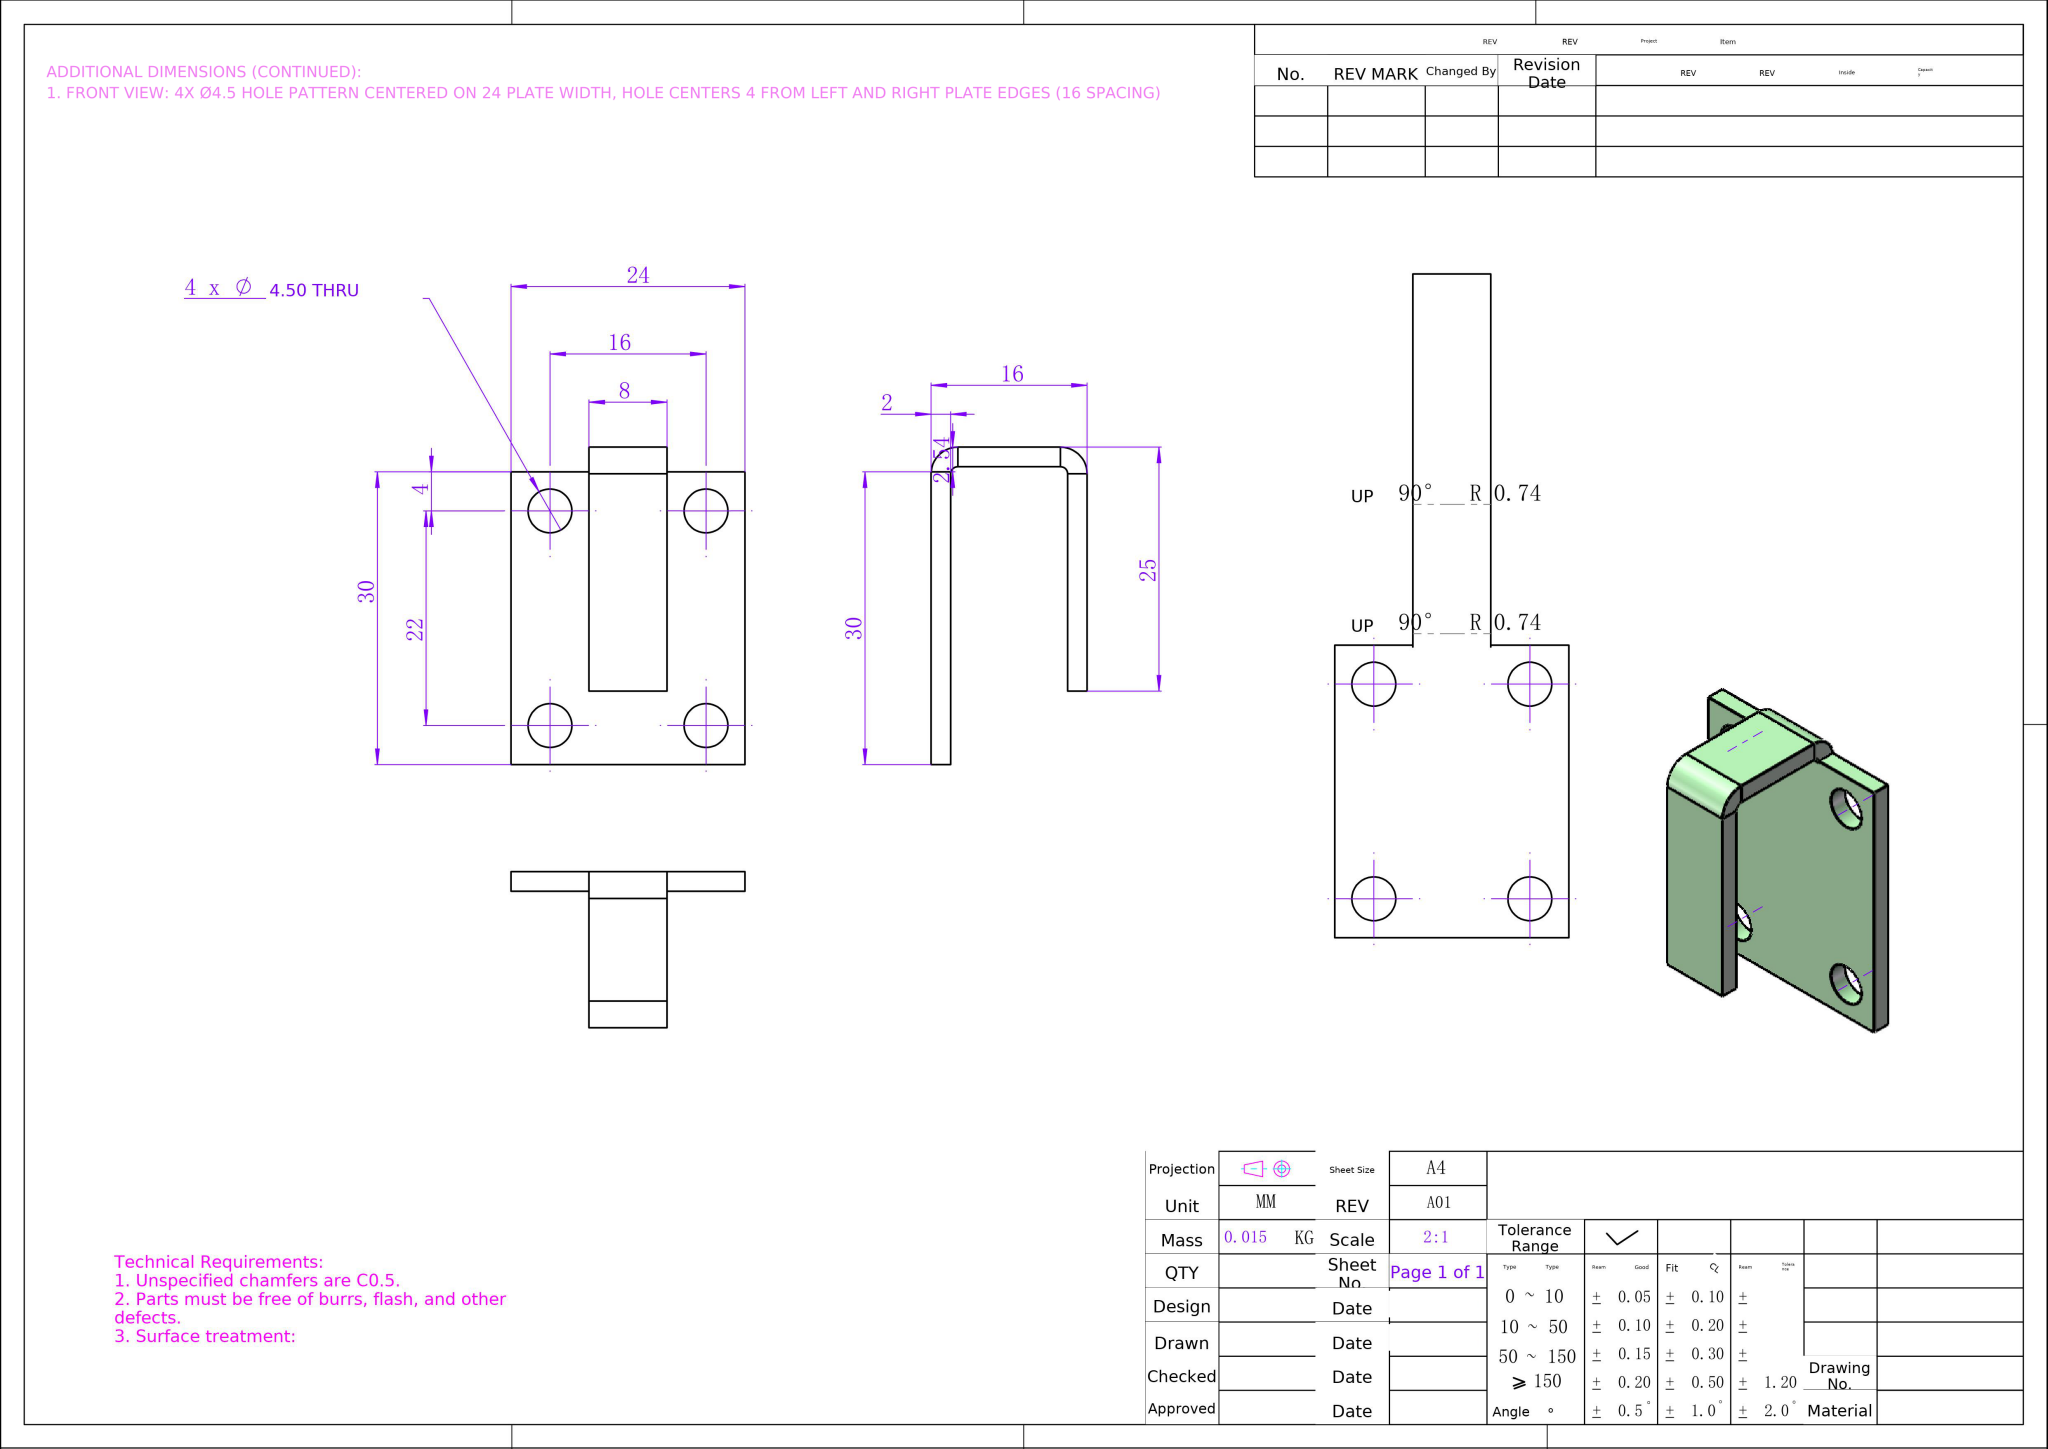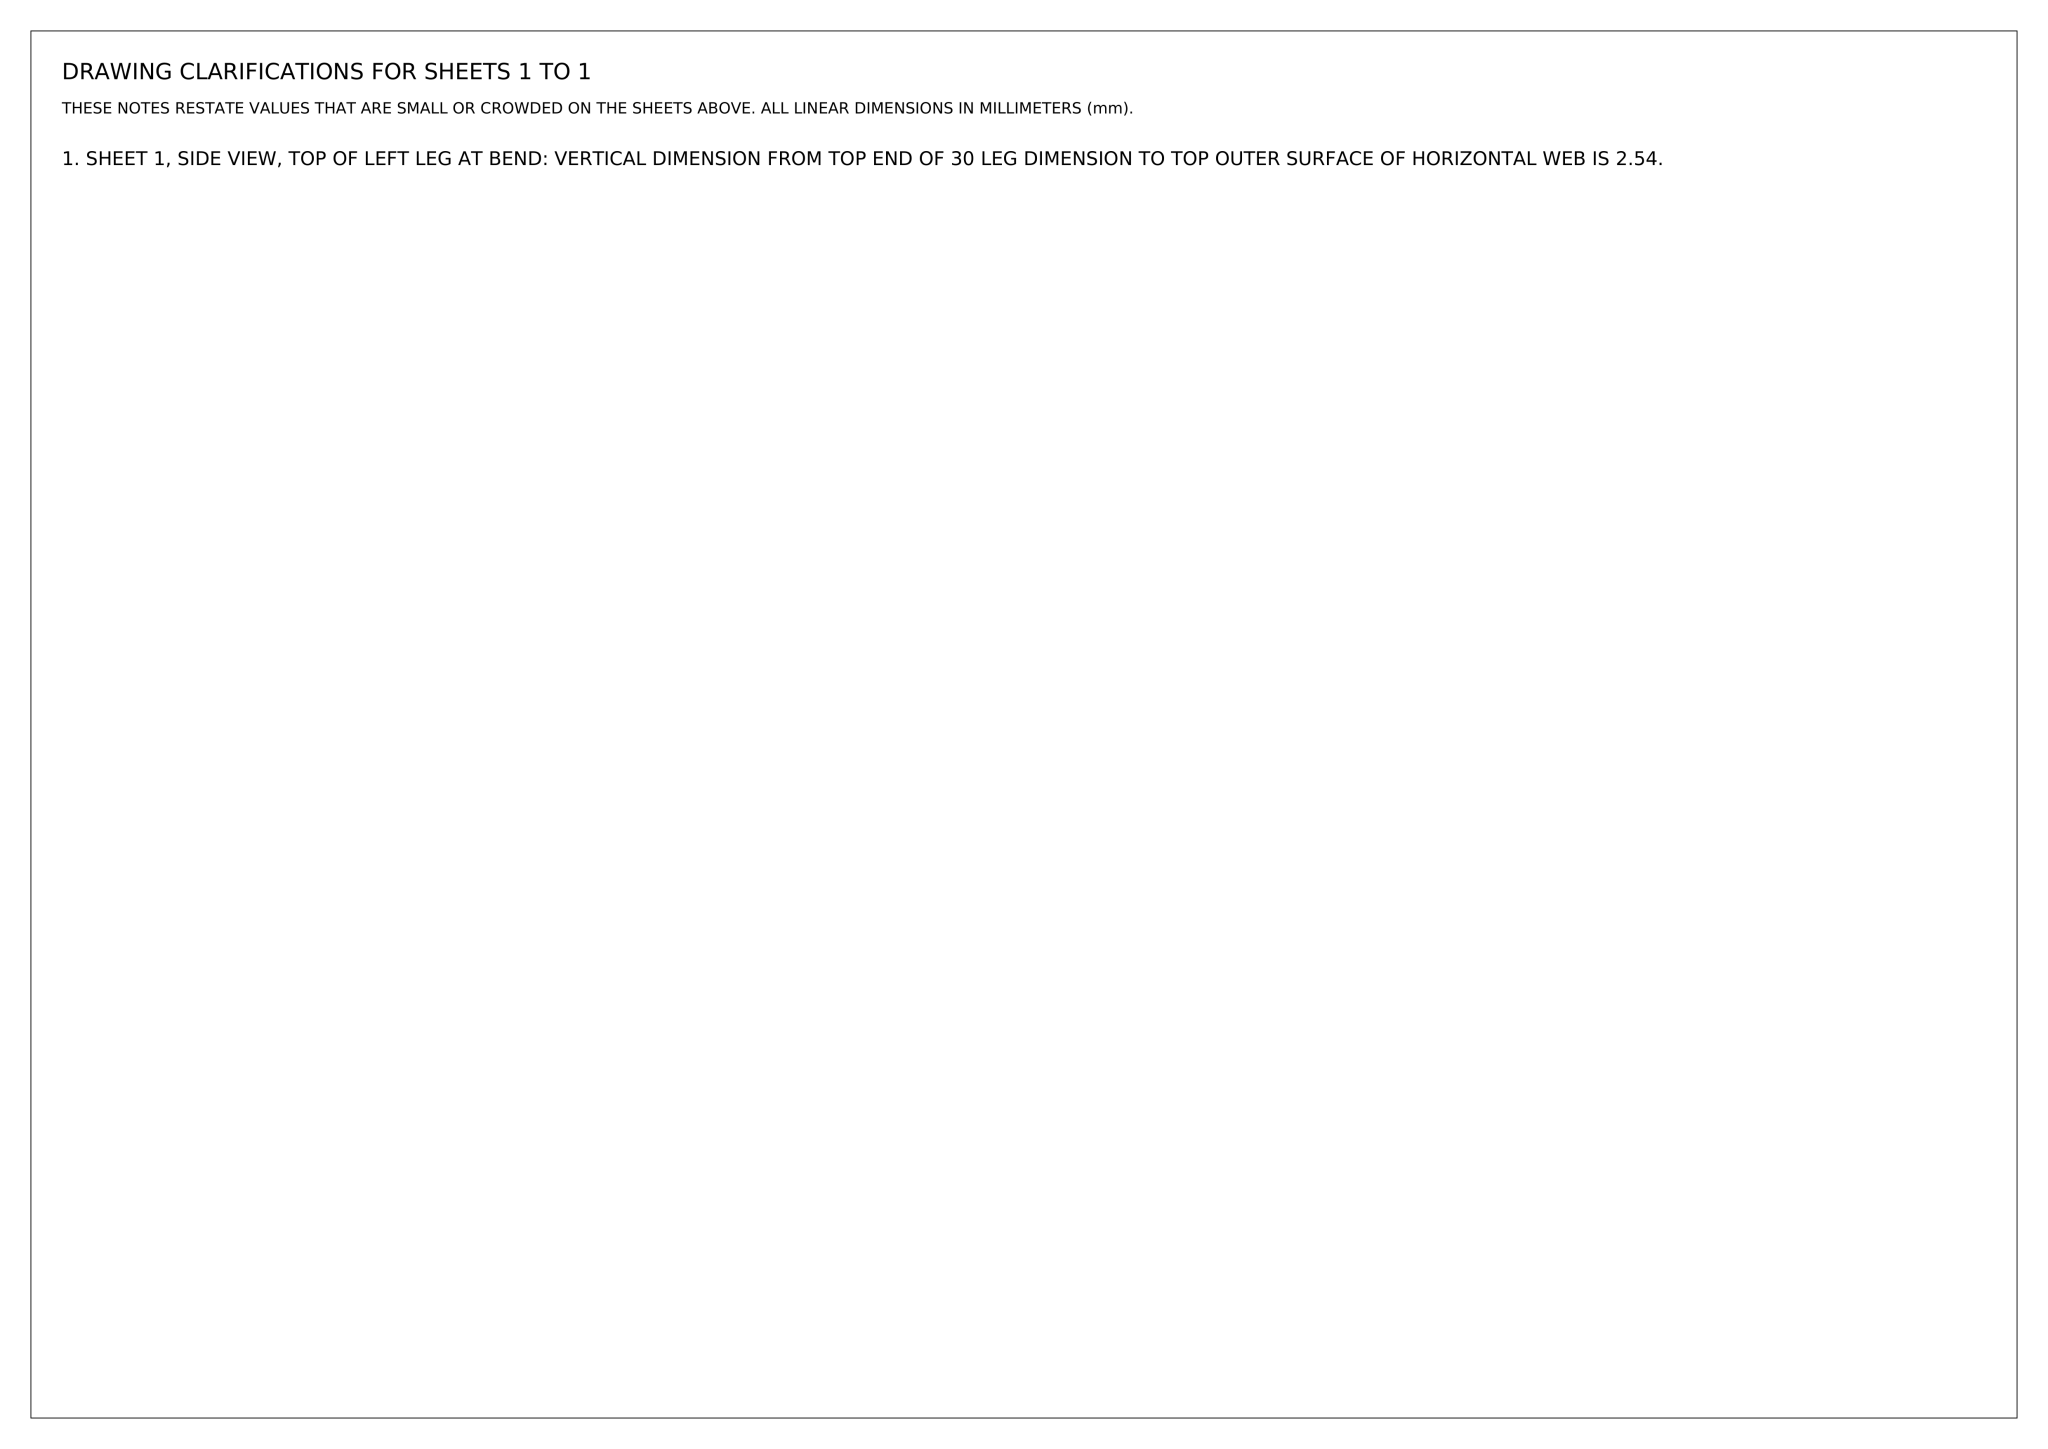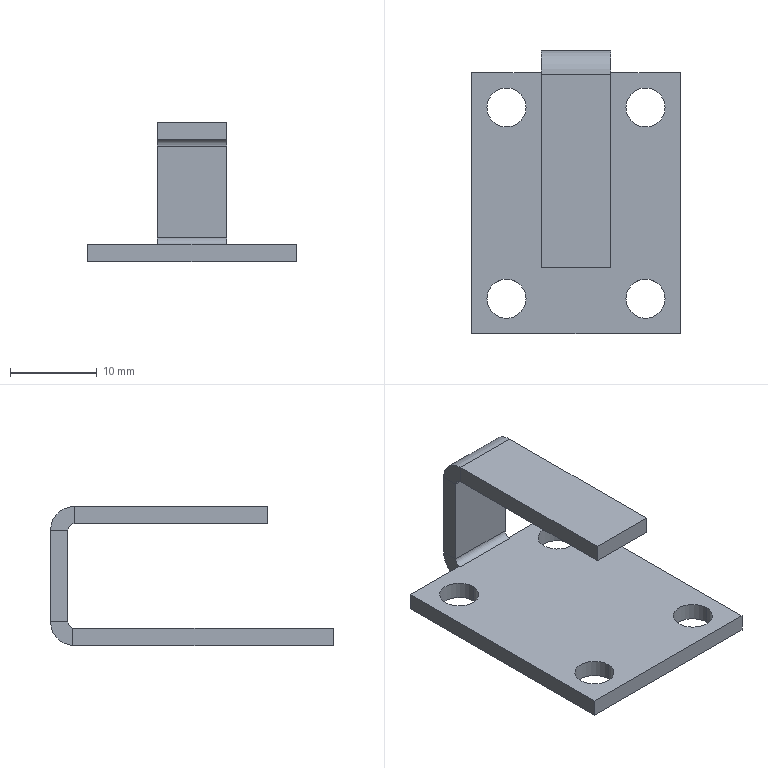Part | NX | mm | 1 solid | 34 faces | box 24 x 32.54 x 16 mm | volume 1921 mm3 | plane 22 | cylinder 12 | commonest cylinder face diameters 4.5 x8 5.473 x2 1.473 x2